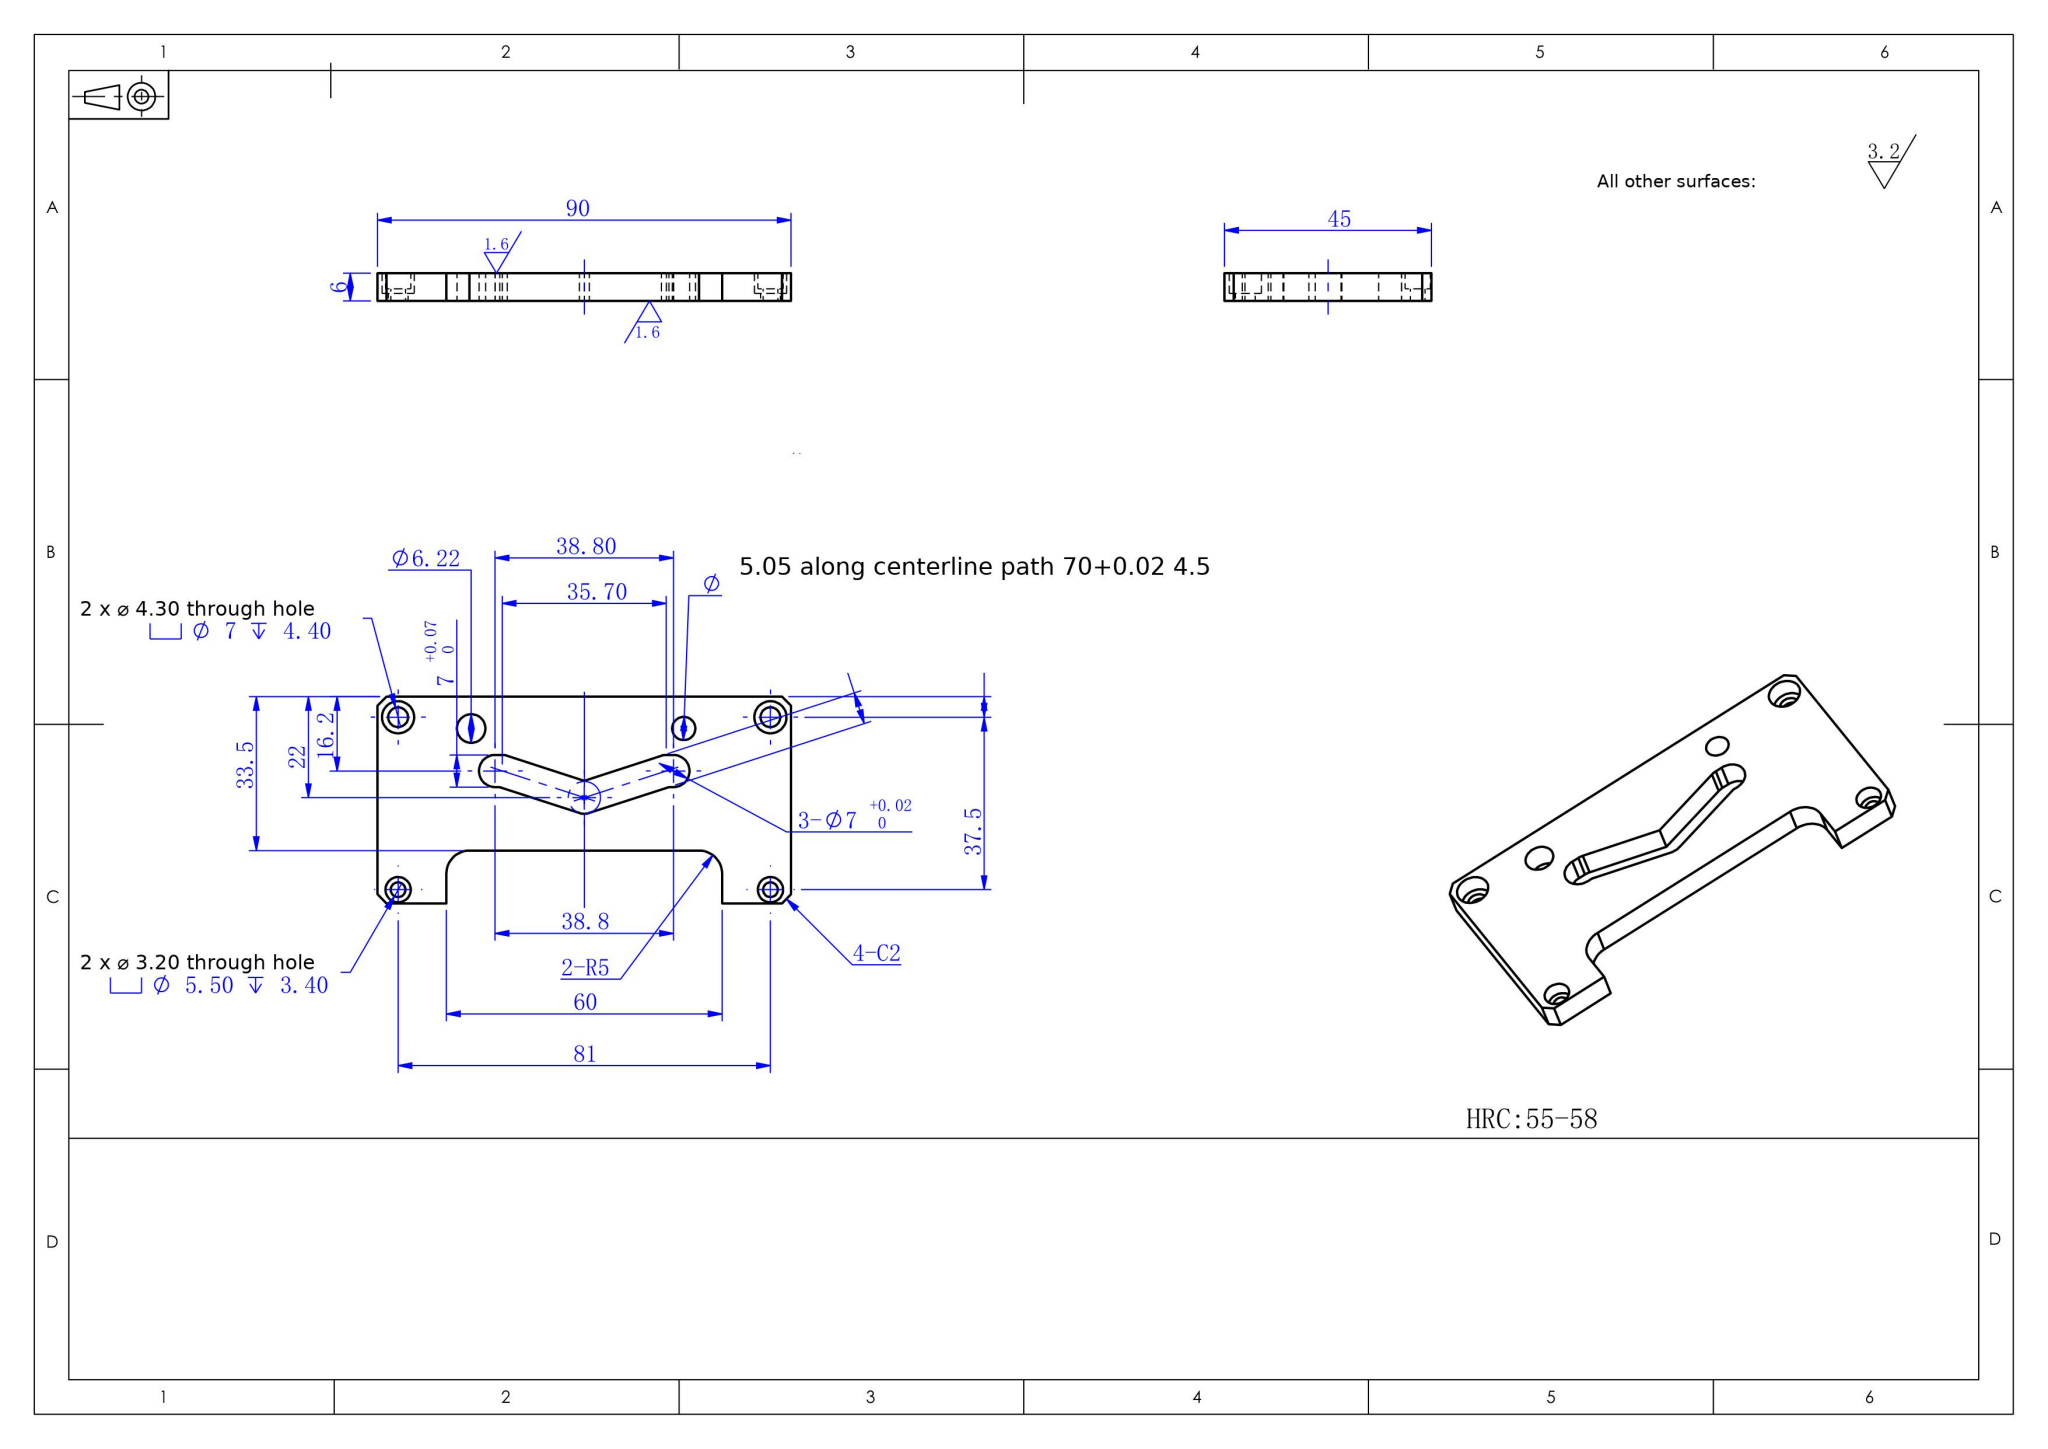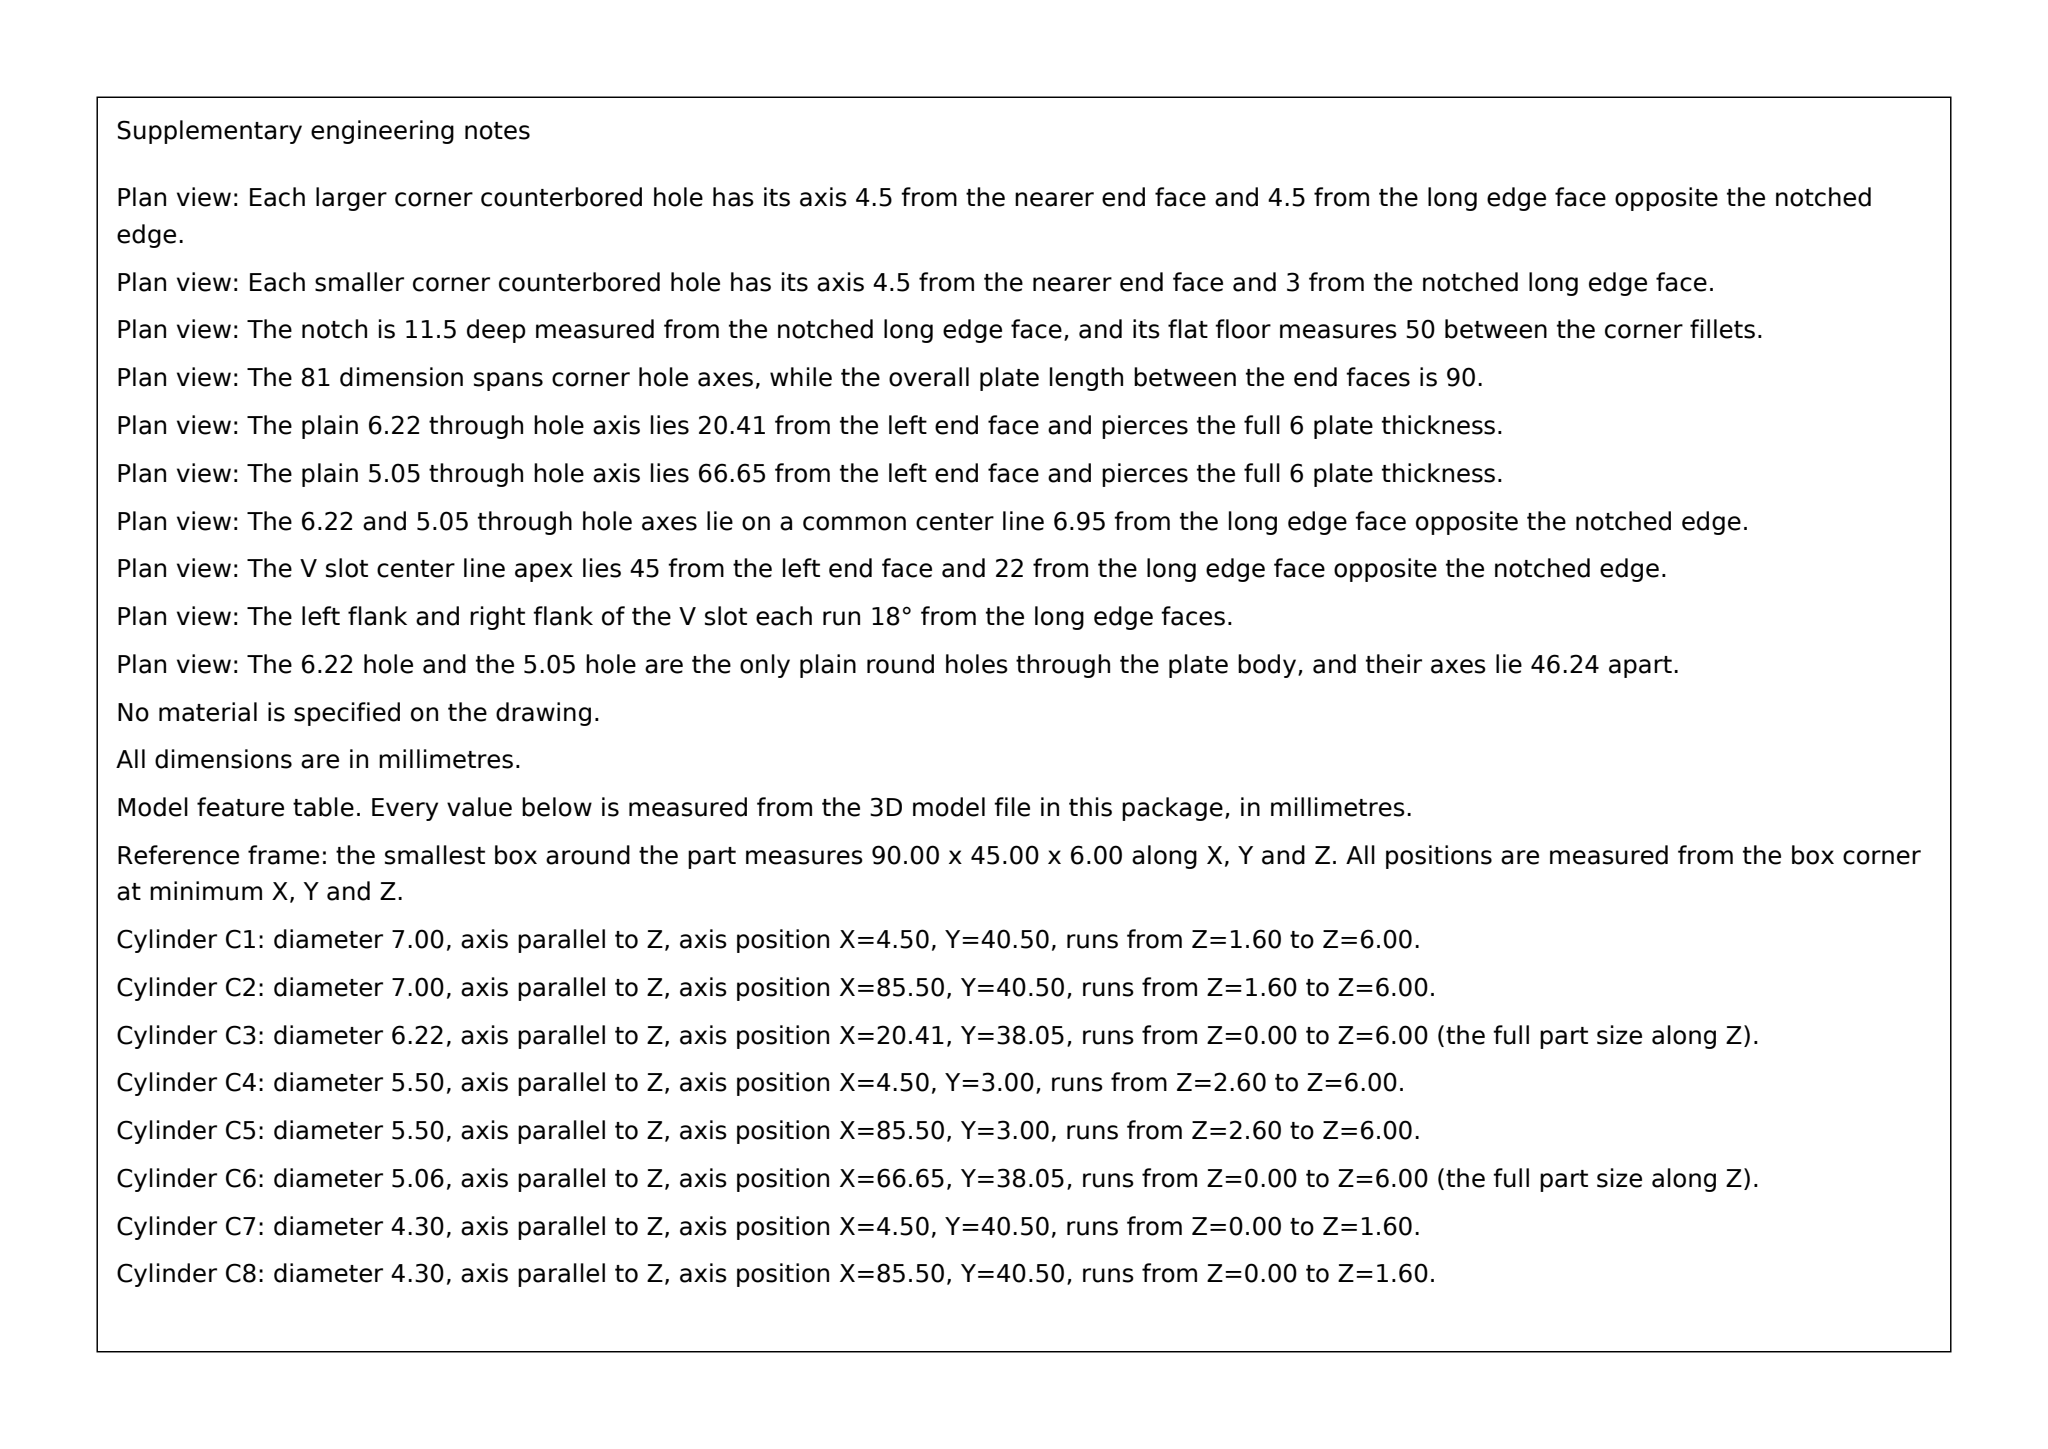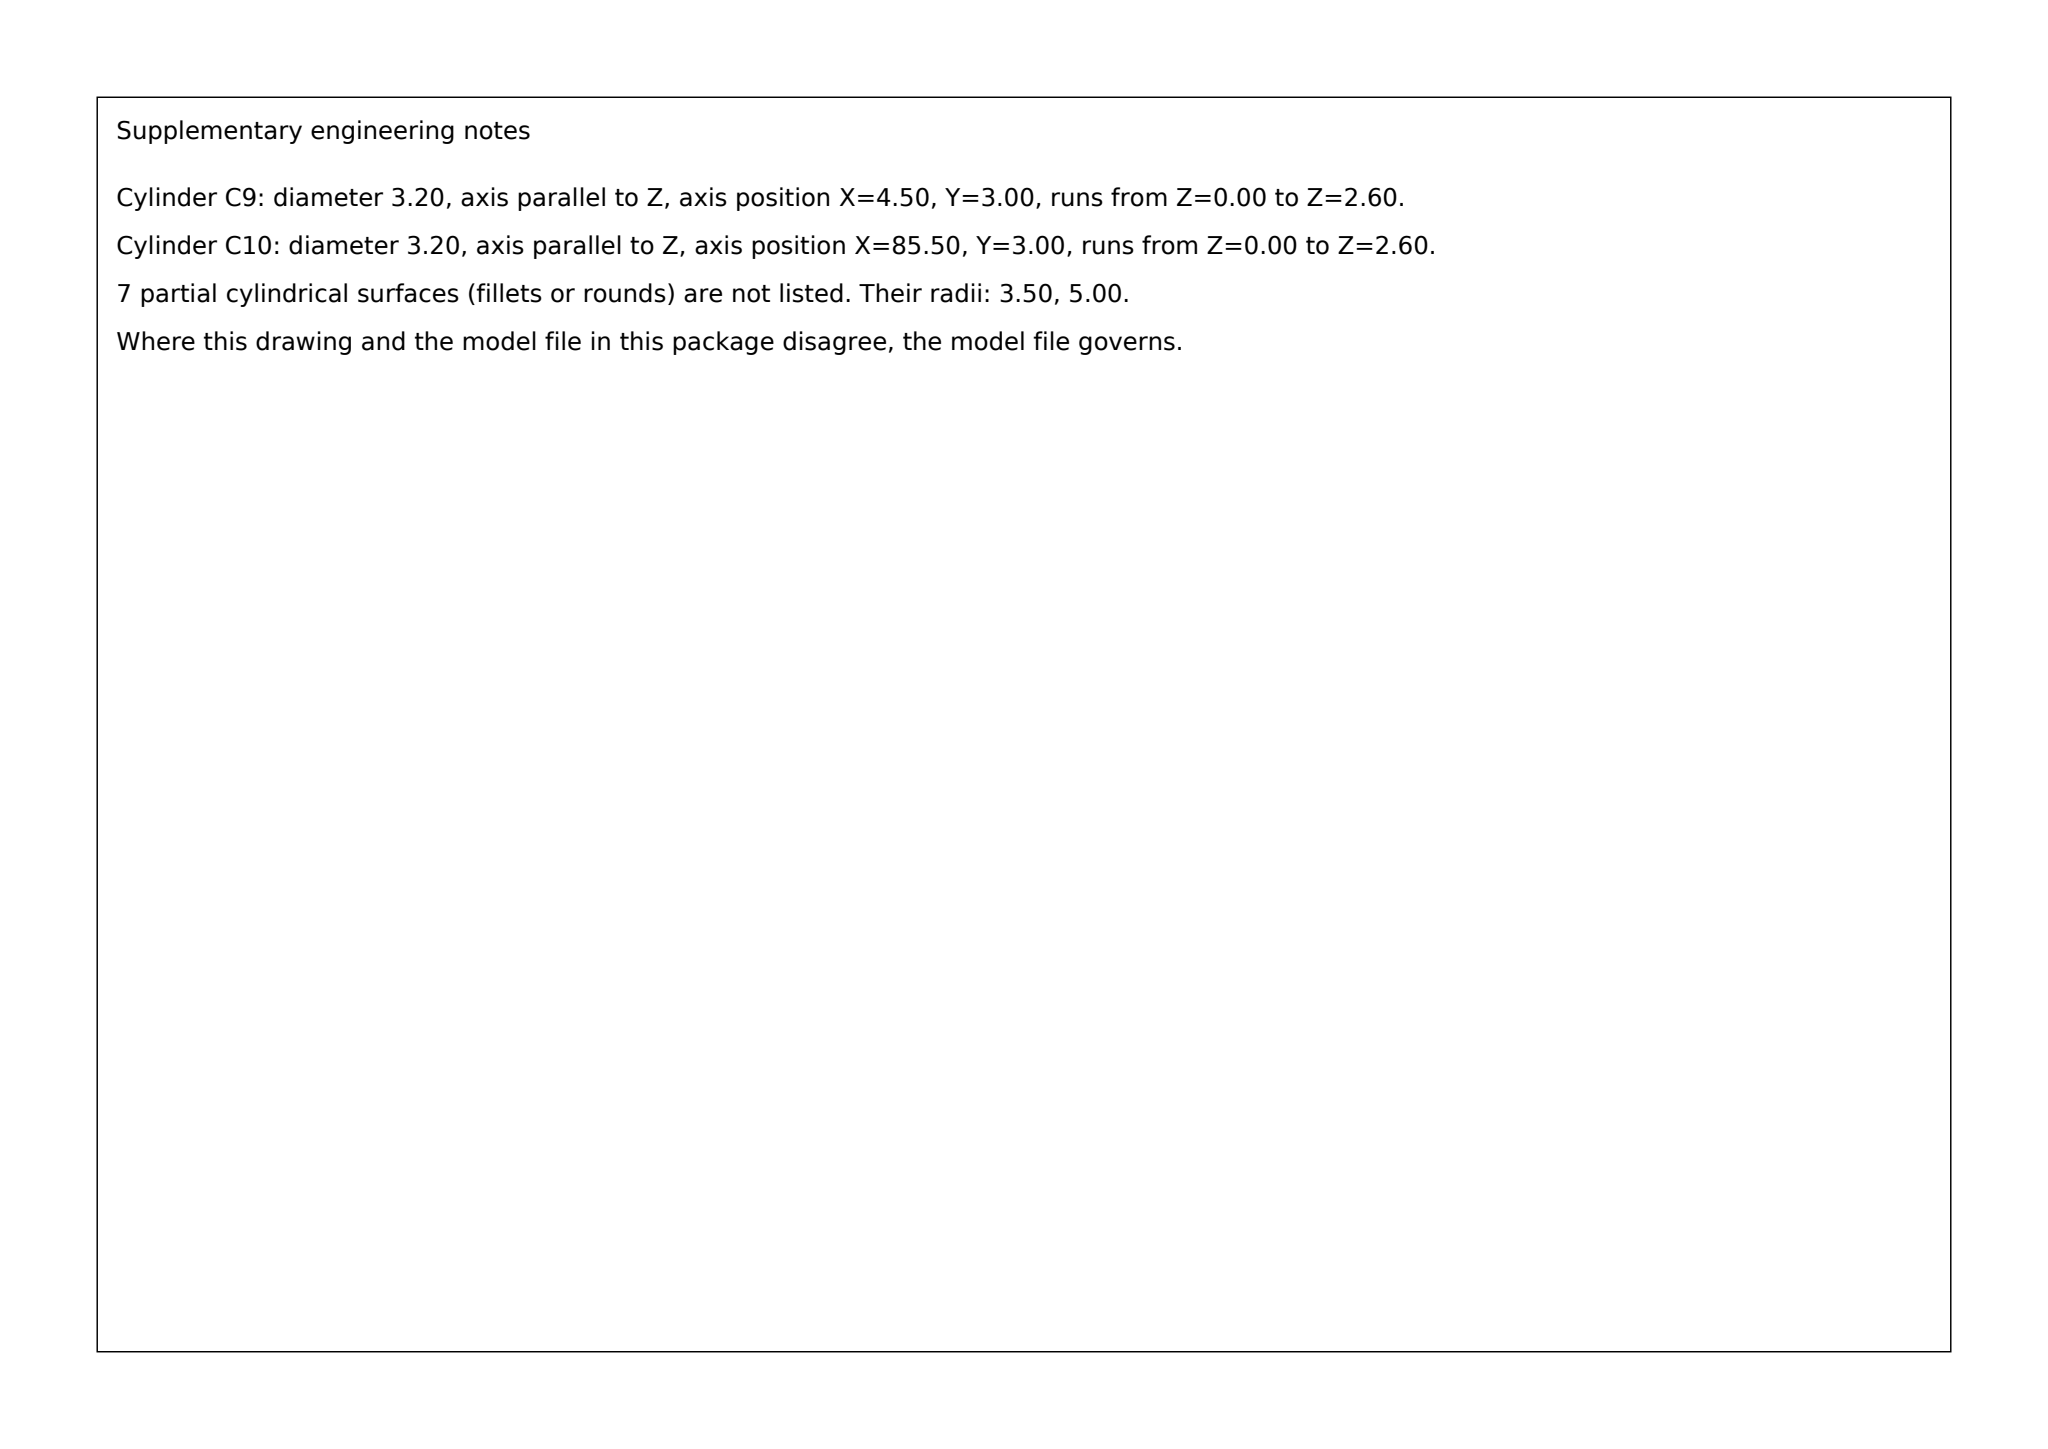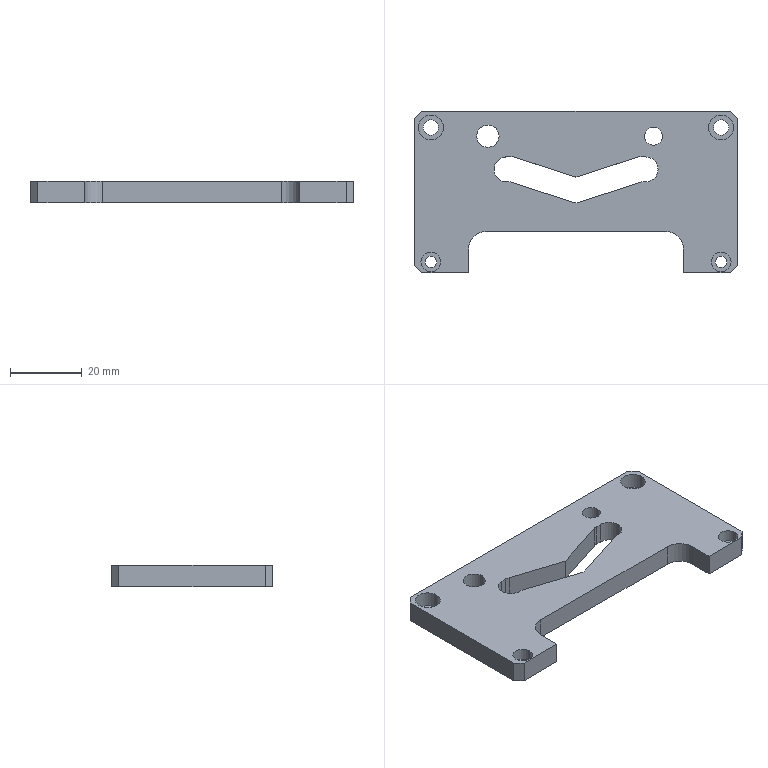Part | SolidWorks | mm | 1 solid | 54 faces | box 90 x 45 x 6 mm | volume 17348 mm3 | cylinder 28 | plane 26 | commonest cylinder face diameters 7 x10 5.5 x4 3.2 x4 4.3 x4 6.222 x2 5.051 x2 10 x2
Drawing notes:
Ø5.05 THRU hole: center located 66.65 from left edge and 38.05 from bottom edge (plate datum = lower-left corner); depth 6.0 = thru. | from the solid: cylinders: [5.051,'z',[66.65,38.05],6.0] with bbox_xyz z=6.0
2X Ø4.30 THRU, CBORE Ø7 DP 4.4: centers at X=4.5 and X=85.5 from left edge, Y=40.5 from bottom edge (4.5 from top edge). | from the solid: cylinders: [4.3,'z',[4.5,40.5],1.6] & [4.3,'z',[85.5,40.5],1.6]; [7.0,'z',[4.5,40.5],4.4] & [7.0,'z',[85.5,40.5],4.4]; bbox y=45.0
2X Ø3.20 THRU, CBORE Ø5.50 DP 3.4: centers at X=4.5 and X=85.5 from left edge, Y=3.0 from bottom edge. | from the solid: cylinders: [3.2,'z',[4.5,3.0],2.6] & [3.2,'z',[85.5,3.0],2.6]; [5.5,'z',[4.5,3.0],3.4] & [5.5,'z',[85.5,3.0],3.4]
Ø6.22 THRU hole: center located 20.41 from left edge and 38.05 from bottom edge (value restored from redacted callout). | from the solid: cylinders: [6.222,'z',[20.41,38.05],6.0]
V-slot: 7.0 wide THRU (6.0 deep), slot end centers at X=25.6 and X=64.4, Y=28.8; vertex center at X=45.0, Y=23.0 from lower-left corner. | from the solid: cylinders: [7.0,'z',[25.6,28.8],6.0], [7.0,'z',[64.4,28.8],6.0], [7.0,'z',[45.0,23.0],6.0]
ALL DIMENSIONS IN MILLIMETERS. Overall plate 90 x 45 x 6. | from the solid: bbox_xyz [90.0,45.0,6.0] in mm
build123d program:
from build123d import *

# Parameters (mm, degrees)
SKETCH1_W                                       = 90
SKETCH1_H                                       = 45
BOSS_EXTRUDE1_DEPTH                             = 6
CUT_EXTRUDE2_DEPTH                              = 139.245
M4_HEX_SOCKET_HEAD_CAP_SCREW_CBORE2_D           = 4.3
M4_HEX_SOCKET_HEAD_CAP_SCREW_CBORE2_CBORE_D     = 7
M4_HEX_SOCKET_HEAD_CAP_SCREW_CBORE2_CBORE_DEPTH = 4.4
M3_HEX_SOCKET_HEAD_CAP_SCREW_CBORE4_D           = 3.2
M3_HEX_SOCKET_HEAD_CAP_SCREW_CBORE4_CBORE_D     = 5.5
M3_HEX_SOCKET_HEAD_CAP_SCREW_CBORE4_CBORE_DEPTH = 3.4
CHAMFER1_SIZE                                   = 2
CUT_EXTRUDE3_DEPTH                              = 139.245
SKETCH17_R                                      = 3.111
SKETCH17_R_2                                    = 2.525
CUT_EXTRUDE4_DEPTH                              = 32


with BuildPart() as part:
    # Sketch1 → Boss-Extrude1 (new body)
    with BuildSketch(Plane.XY):
        with Locations((-79.468, 37.362)):
            Rectangle(SKETCH1_W, SKETCH1_H)
    extrude(amount=BOSS_EXTRUDE1_DEPTH)

    # Sketch5 → Cut-Extrude2 (cut, through all)
    with BuildSketch(Plane.XY.offset(6)):
        with BuildLine():
            Line((-109.468, 14.862), (-49.468, 14.862))
            Line((-49.468, 14.862), (-49.468, 21.362))
            ThreePointArc((-49.468, 21.362), (-50.933, 24.897), (-54.468, 26.362))
            Line((-54.468, 26.362), (-104.468, 26.362))
            ThreePointArc((-104.468, 26.362), (-108.004, 24.897), (-109.468, 21.362))
            Line((-109.468, 21.362), (-109.468, 14.862))
        make_face()
    extrude(amount=-CUT_EXTRUDE2_DEPTH, mode=Mode.SUBTRACT)

    # M4 Hex Socket Head Cap Screw CBORE2 (through all)
    with Locations(Plane.XY.offset(6)):
        with Locations((-119.968, 55.362), (-38.968, 55.362)):
            CounterBoreHole(M4_HEX_SOCKET_HEAD_CAP_SCREW_CBORE2_D / 2, M4_HEX_SOCKET_HEAD_CAP_SCREW_CBORE2_CBORE_D / 2, M4_HEX_SOCKET_HEAD_CAP_SCREW_CBORE2_CBORE_DEPTH)

    # M3 Hex Socket Head Cap Screw CBORE4 (through all)
    with Locations(Plane.XY.offset(6)):
        with Locations((-119.968, 17.862), (-38.968, 17.862)):
            CounterBoreHole(M3_HEX_SOCKET_HEAD_CAP_SCREW_CBORE4_D / 2, M3_HEX_SOCKET_HEAD_CAP_SCREW_CBORE4_CBORE_D / 2, M3_HEX_SOCKET_HEAD_CAP_SCREW_CBORE4_CBORE_DEPTH)

    # Chamfer1
    chamfer1_edges = [part.edges().sort_by_distance(p)[0] for p in [
        (-124.468, 59.862, 3),
        (-34.468, 59.862, 3),
        (-34.468, 14.862, 3),
        (-124.468, 14.862, 3),
    ]]
    chamfer(chamfer1_edges, length=CHAMFER1_SIZE)

    # Sketch16 → Cut-Extrude3 (cut, through all)
    with BuildSketch(Plane.XY.offset(6)):
        with BuildLine():
            Line((-80.55, 41.19), (-62.7, 46.99))
            ThreePointArc((-62.7, 46.99), (-62.166, 47.118), (-61.618, 47.162))
            Line((-61.618, 47.162), (-60.066, 47.162))
            ThreePointArc((-60.066, 47.162), (-56.566, 43.662), (-60.066, 40.162))
            Line((-60.066, 40.162), (-61.064, 40.162))
            Line((-61.064, 40.162), (-78.387, 34.533))
            ThreePointArc((-78.387, 34.533), (-82.797, 36.78), (-80.55, 41.19))
        make_face()
    cut_extrude3 = extrude(amount=-CUT_EXTRUDE3_DEPTH, mode=Mode.SUBTRACT)

    # Mirror1: Cut-Extrude3 across plane
    add(cut_extrude3.mirror(Plane(origin=(-79.468, 0, 0), x_dir=(0, 0, 1), z_dir=(1, 0, 0))), mode=Mode.SUBTRACT)

    # Sketch17 → Cut-Extrude4 (cut)
    with BuildSketch(Plane.XY.offset(6)):
        with Locations((-104.061, 52.914)):
            Circle(SKETCH17_R)
        with Locations((-57.82, 52.914)):
            Circle(SKETCH17_R_2)
    extrude(amount=-CUT_EXTRUDE4_DEPTH, mode=Mode.SUBTRACT)


solid = part.part